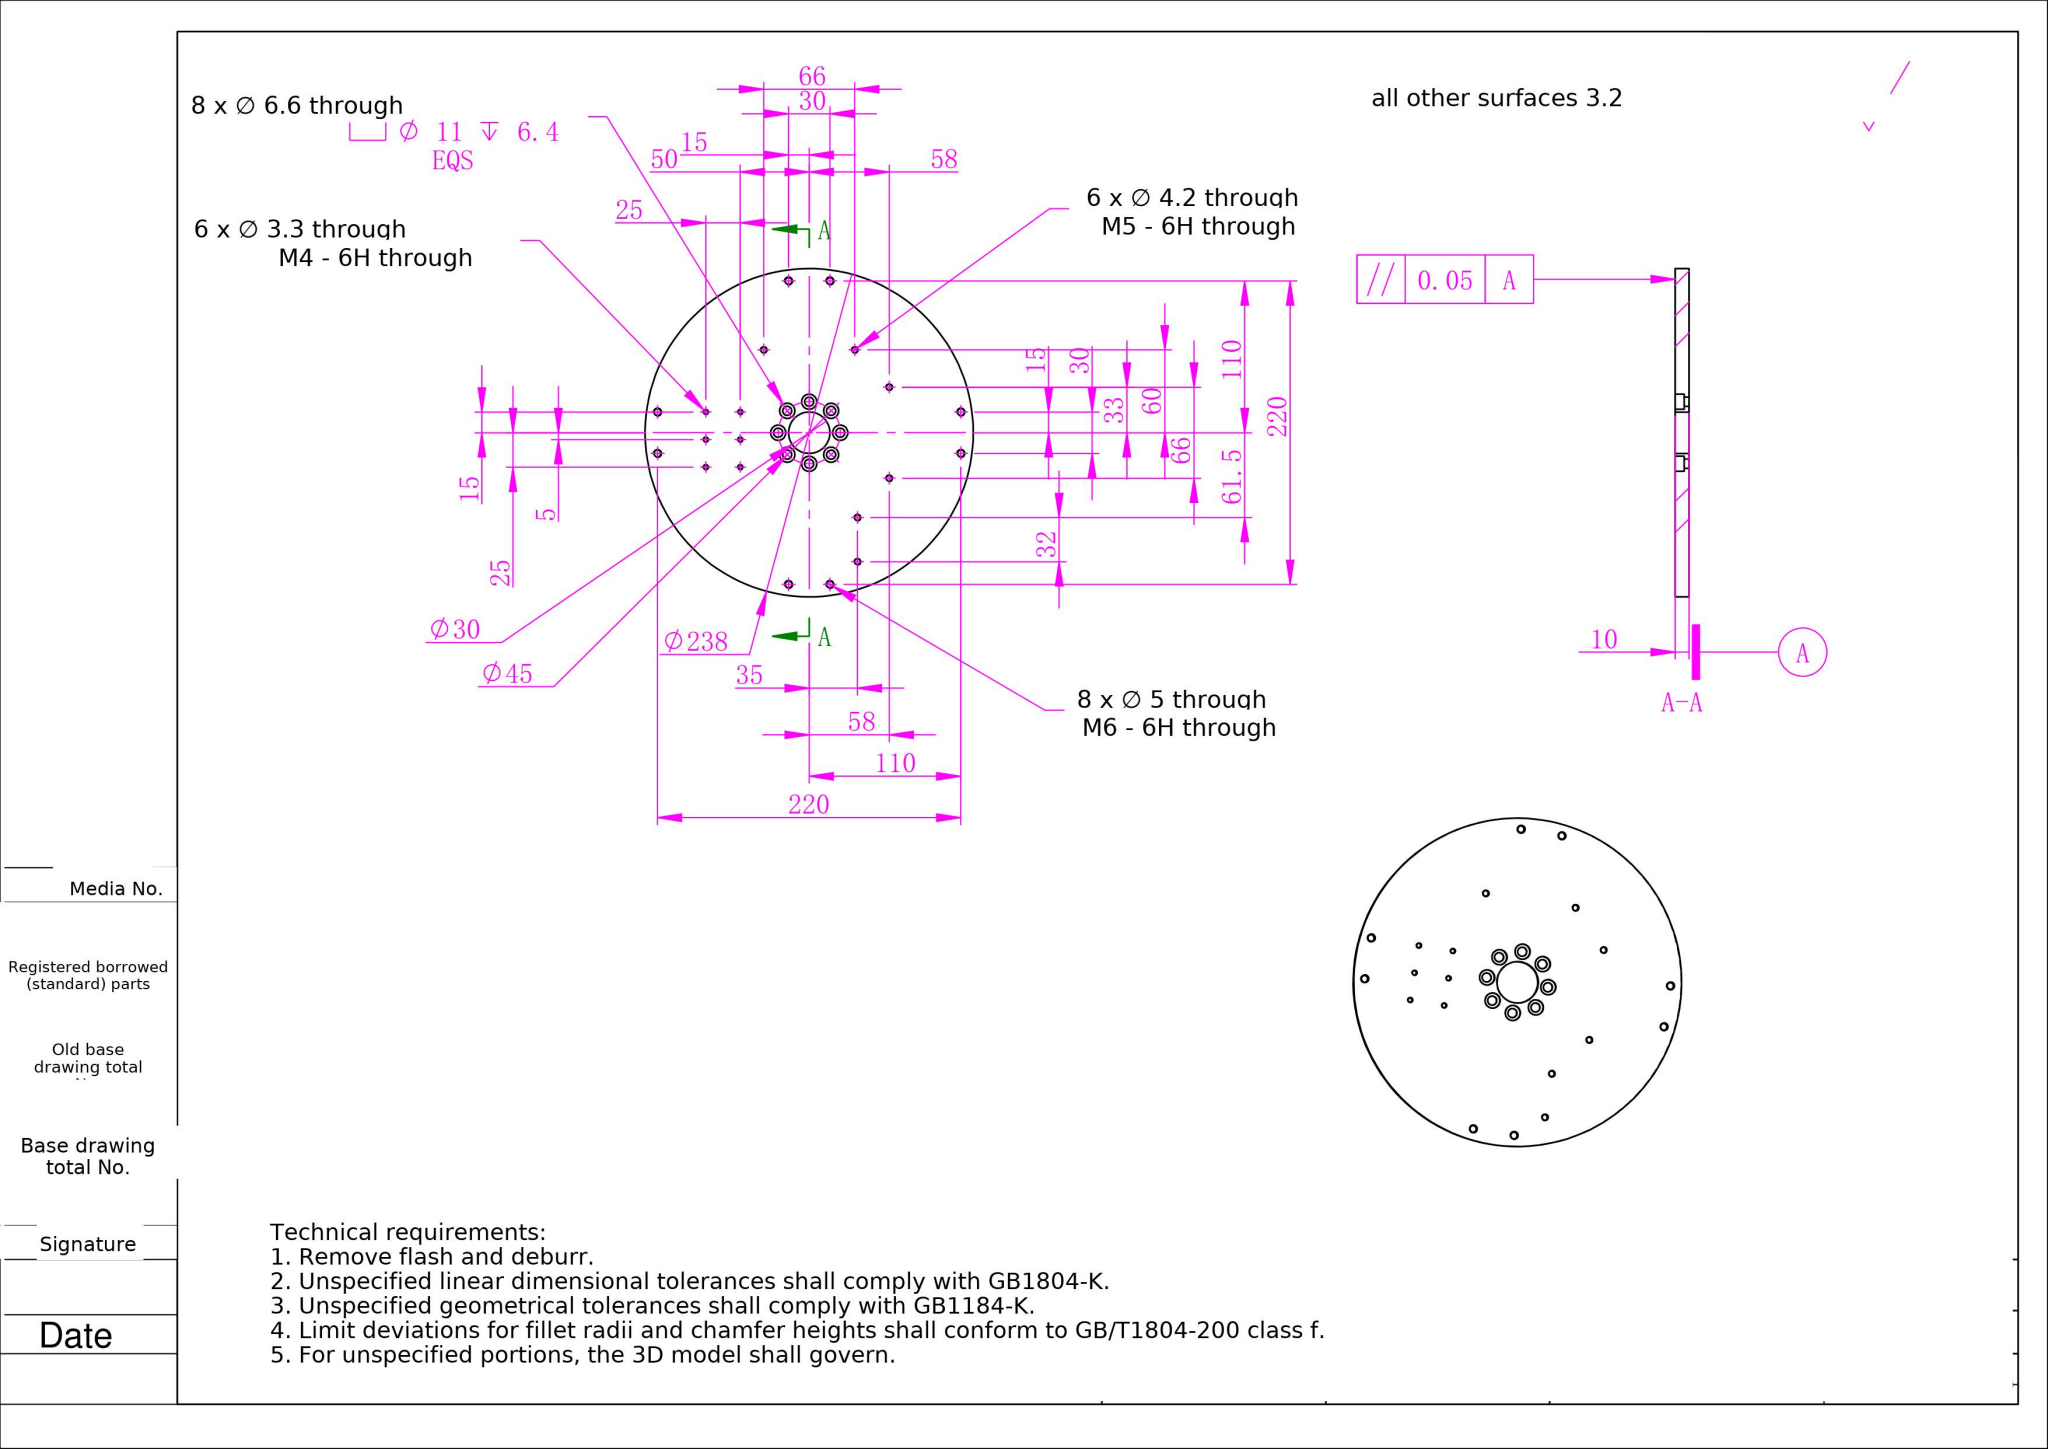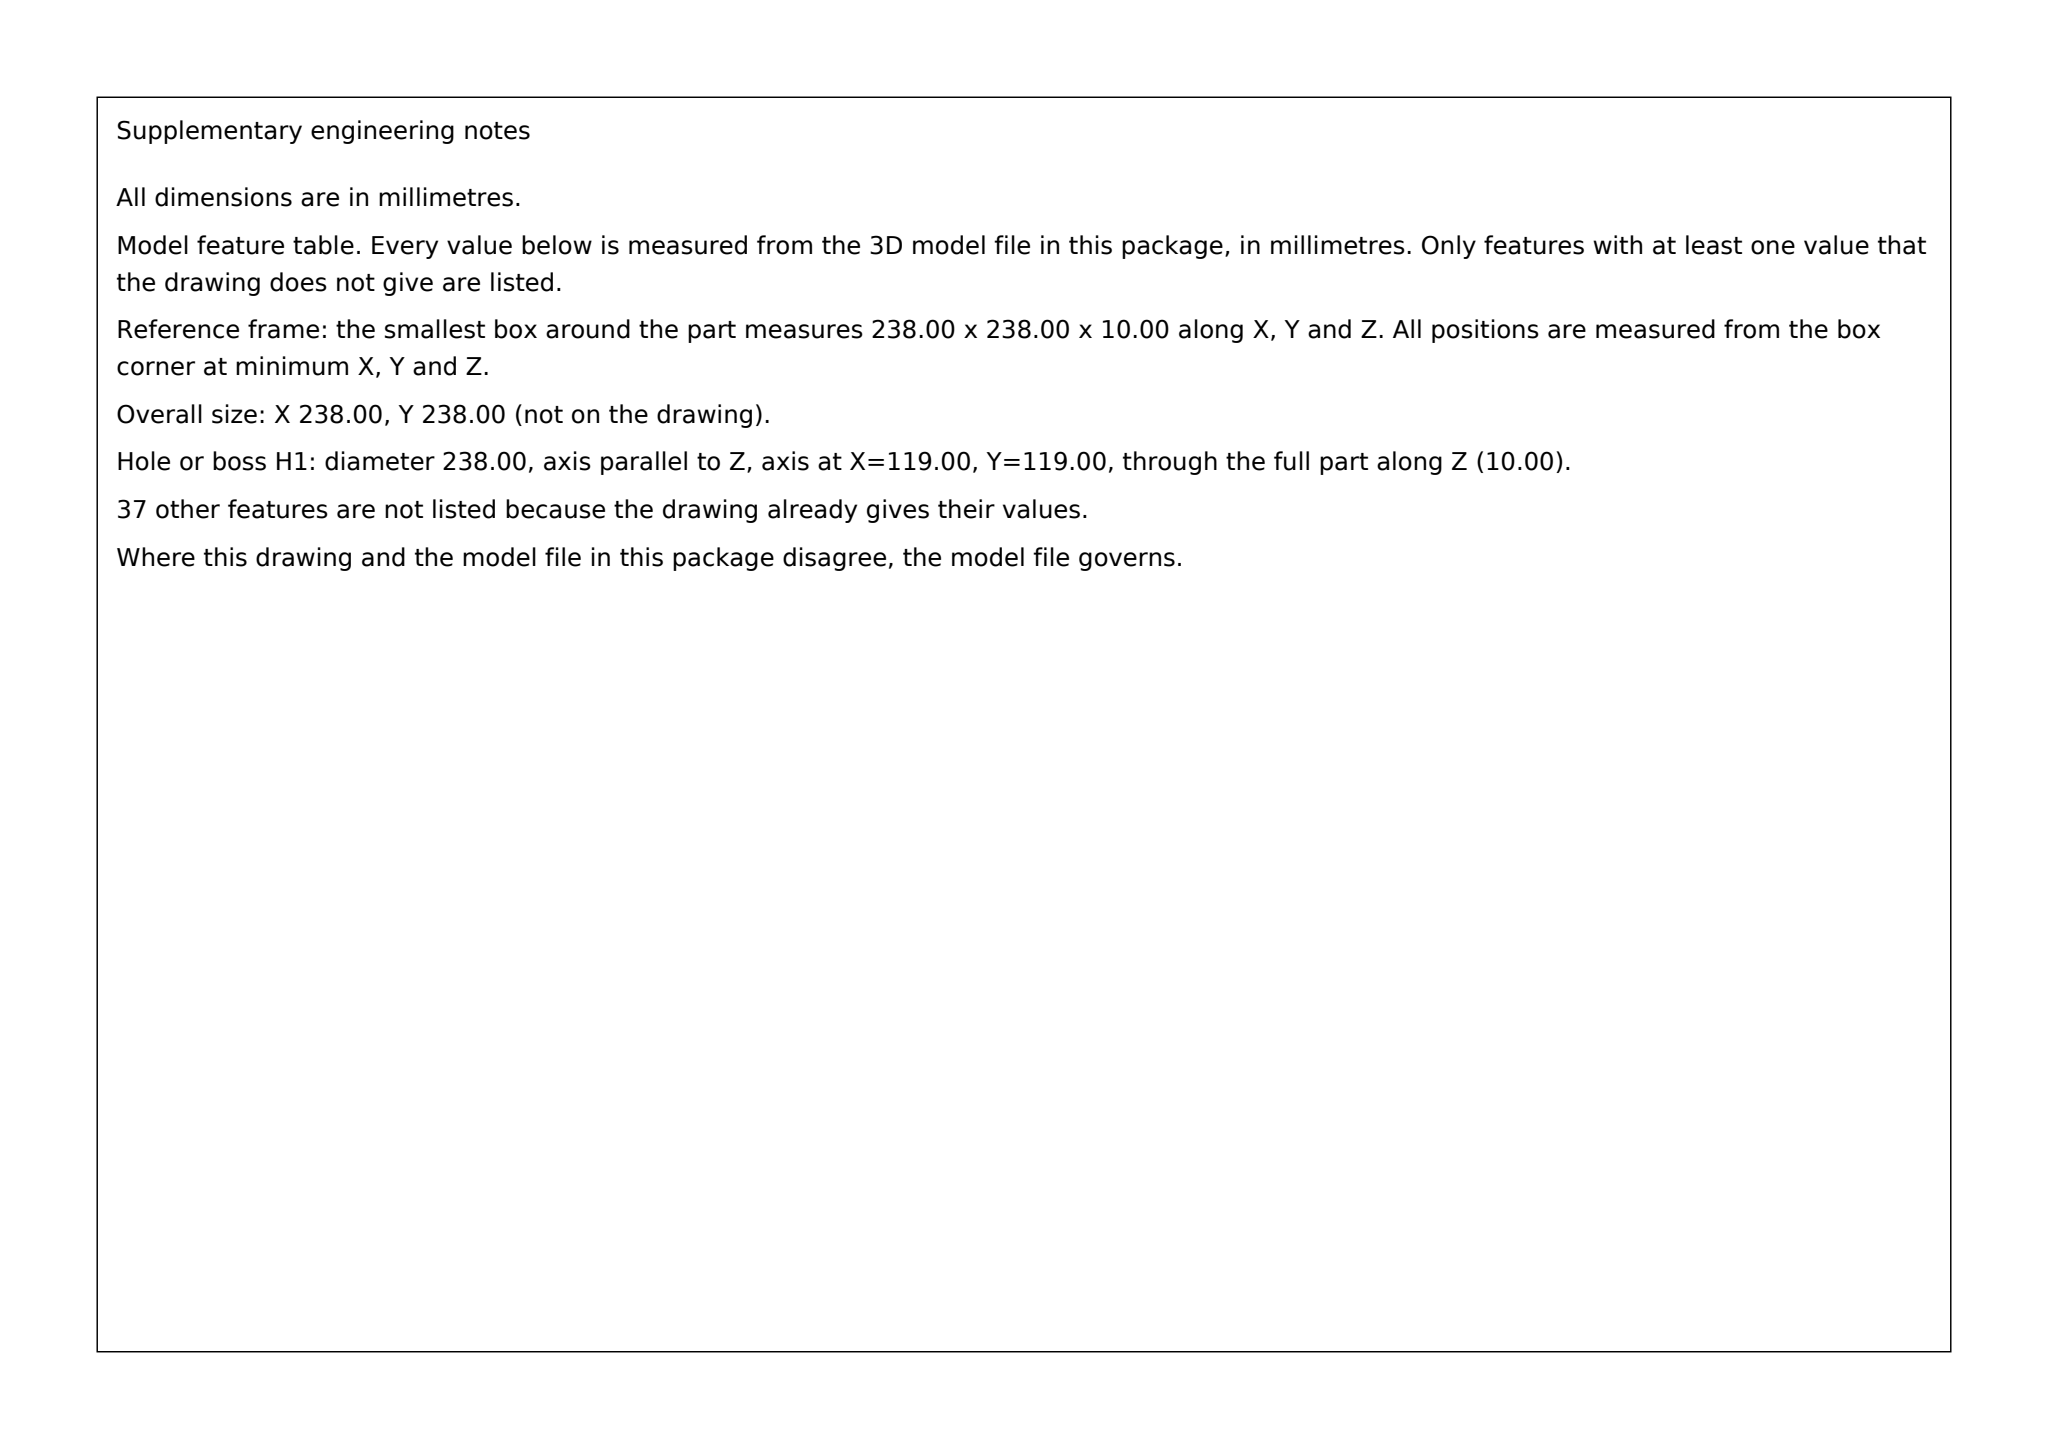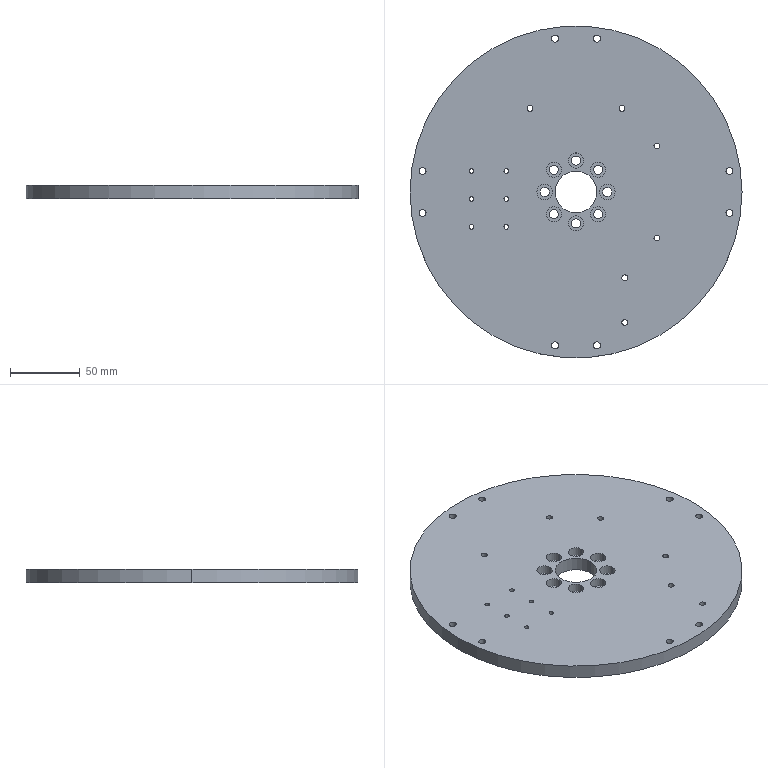Part | SolidWorks | mm | 1 solid | 86 faces | box 238 x 238 x 10 mm | volume 429046 mm3 | cylinder 76 | plane 10 | commonest cylinder face diameters 5 x16 11 x16 6.6 x16 4.2 x12 3.3 x12 30 x2 238 x2
build123d program:
from build123d import *

# Parameters (mm, degrees)
SKETCH1_R                                       = 119
BOSS_EXTRUDE1_DEPTH                             = 5
SKETCH2_R                                       = 15
CUT_EXTRUDE1_DEPTH                              = 169.588
M6_HEX_SOCKET_HEAD_CAP_SCREW_CBORE1_D           = 6.6
M6_HEX_SOCKET_HEAD_CAP_SCREW_CBORE1_CBORE_D     = 11
M6_HEX_SOCKET_HEAD_CAP_SCREW_CBORE1_CBORE_DEPTH = 6.4
CIRPATTERN1_COUNT                               = 8
M6_TAPPED_HOLE1_D                               = 5
CIRPATTERN2_COUNT                               = 4
M5_TAPPED_HOLE2_D                               = 4.2
M4_TAPPED_HOLE1_D                               = 3.3
M5_TAPPED_HOLE3_D                               = 4.2
M5_TAPPED_HOLE4_D                               = 4.2


with BuildPart() as part:
    # Sketch1 → Boss-Extrude1 (new, symmetric)
    with BuildSketch(Plane.XY):
        Circle(SKETCH1_R)
    extrude(amount=BOSS_EXTRUDE1_DEPTH, both=True)

    # Sketch2 → Cut-Extrude1 (cut, through all)
    with BuildSketch(Plane.XY.offset(5)):
        Circle(SKETCH2_R)
    extrude(amount=-CUT_EXTRUDE1_DEPTH, mode=Mode.SUBTRACT)

    # M6 Hex Socket Head Cap Screw CBORE1 (through all)
    with Locations(Plane.XY.offset(5)):
        with Locations((0, 22.5)):
            m6_hex_socket_head_cap_screw_cbore1 = CounterBoreHole(M6_HEX_SOCKET_HEAD_CAP_SCREW_CBORE1_D / 2, M6_HEX_SOCKET_HEAD_CAP_SCREW_CBORE1_CBORE_D / 2, M6_HEX_SOCKET_HEAD_CAP_SCREW_CBORE1_CBORE_DEPTH)

    # CirPattern1: M6 Hex Socket Head Cap Screw CBORE1 ×8 about axis
    cirpattern1_axis = Axis((0, 0, 0), (0, 0, 1))
    for i in range(1, CIRPATTERN1_COUNT):
        add(m6_hex_socket_head_cap_screw_cbore1.rotate(cirpattern1_axis, i * 360 / CIRPATTERN1_COUNT), mode=Mode.SUBTRACT)

    # M6 Tapped Hole1 (through all)
    with Locations(Plane.XY.offset(5)):
        with Locations((-15, 110), (15, 110)):
            m6_tapped_hole1 = Hole(M6_TAPPED_HOLE1_D / 2)

    # CirPattern2: M6 Tapped Hole1 ×4 about axis
    cirpattern2_axis = Axis((0, 0, 0), (0, 0, 1))
    for i in range(1, CIRPATTERN2_COUNT):
        add(m6_tapped_hole1.rotate(cirpattern2_axis, i * 360 / CIRPATTERN2_COUNT), mode=Mode.SUBTRACT)

    # M5 Tapped Hole2 (through all)
    with Locations(Plane.XY.offset(5)):
        with Locations((-33, 60), (33, 60)):
            Hole(M5_TAPPED_HOLE2_D / 2)

    # M4 Tapped Hole1 (through all)
    with Locations(Plane.XY.offset(5)):
        with Locations((-50, -25), (-50, 15), (-75, 15), (-75, -5), (-50, -5), (-75, -25)):
            Hole(M4_TAPPED_HOLE1_D / 2)

    # M5 Tapped Hole3 (through all)
    with Locations(Plane.XY.offset(5)):
        with Locations((35, -61.5), (35, -93.5)):
            Hole(M5_TAPPED_HOLE3_D / 2)

    # M5 Tapped Hole4 (through all)
    with Locations(Plane.XY.offset(5)):
        with Locations((58, 33), (58, -33)):
            Hole(M5_TAPPED_HOLE4_D / 2)


solid = part.part